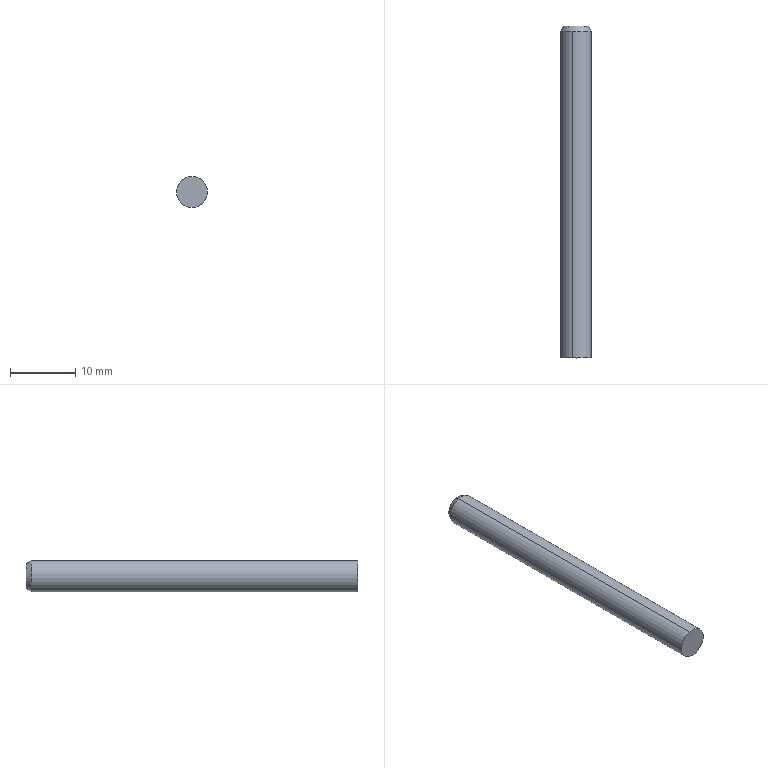Component | SolidWorks | Imported2-1 | 1 solid | 6 faces | box 4.75 x 50.8 x 4.75 mm | volume 898 mm3 | cone 2 | cylinder 2 | plane 2 | commonest cylinder face diameters 4.75 x2
STEP:
#1=CARTESIAN_POINT('',(-8.215,7.373,9.956));
#2=VERTEX_POINT('',#1);
#3=CARTESIAN_POINT('',(-8.178,7.373,9.809));
#4=VERTEX_POINT('',#3);
#5=CARTESIAN_POINT('',(-8.196,7.373,9.883));
#6=DIRECTION('',(0.,1.,-0.));
#7=DIRECTION('',(-0.2492,0.,0.9685));
#8=AXIS2_PLACEMENT_3D('',#5,#6,#7);
#9=CIRCLE('',#8,0.07546);
#10=EDGE_CURVE('',#2,#4,#9,.T.);
#11=ORIENTED_EDGE('',*,*,#10,.F.);
#12=CARTESIAN_POINT('',(-8.22,7.342,9.973));
#13=VERTEX_POINT('',#12);
#14=CARTESIAN_POINT('',(-8.215,7.373,9.956));
#15=DIRECTION('',(-0.1246,-0.866,0.4842));
#16=VECTOR('',#15,39.37);
#17=LINE('',#14,#16);
#18=EDGE_CURVE('',#2,#13,#17,.T.);
#19=ORIENTED_EDGE('',*,*,#18,.T.);
#20=CARTESIAN_POINT('',(-8.173,7.342,9.792));
#21=VERTEX_POINT('',#20);
#22=CARTESIAN_POINT('',(-8.196,7.342,9.883));
#23=DIRECTION('',(-0.,-1.,0.));
#24=DIRECTION('',(-0.2492,0.,0.9685));
#25=AXIS2_PLACEMENT_3D('',#22,#23,#24);
#26=CIRCLE('',#25,0.0935);
#27=EDGE_CURVE('',#21,#13,#26,.T.);
#28=ORIENTED_EDGE('',*,*,#27,.F.);
#29=CARTESIAN_POINT('',(-8.178,7.373,9.809));
#30=DIRECTION('',(0.1246,-0.866,-0.4842));
#31=VECTOR('',#30,39.37);
#32=LINE('',#29,#31);
#33=EDGE_CURVE('',#4,#21,#32,.T.);
#34=ORIENTED_EDGE('',*,*,#33,.F.);
#35=EDGE_LOOP('',(#11,#19,#28,#34));
#36=FACE_OUTER_BOUND('',#35,.T.);
#37=CARTESIAN_POINT('',(-8.196,7.373,9.883));
#38=DIRECTION('',(-0.,-1.,0.));
#39=DIRECTION('',(0.2492,0.,-0.9685));
#40=AXIS2_PLACEMENT_3D('',#37,#38,#39);
#41=CONICAL_SURFACE('',#40,0.07546,0.5236);
#42=ADVANCED_FACE('',(#36),#41,.T.);
#43=ORIENTED_EDGE('',*,*,#27,.T.);
#44=CARTESIAN_POINT('',(-8.22,5.373,9.973));
#45=VERTEX_POINT('',#44);
#46=CARTESIAN_POINT('',(-8.22,7.373,9.973));
#47=DIRECTION('',(-0.,-1.,0.));
#48=VECTOR('',#47,39.37);
#49=LINE('',#46,#48);
#50=EDGE_CURVE('',#13,#45,#49,.T.);
#51=ORIENTED_EDGE('',*,*,#50,.T.);
#52=CARTESIAN_POINT('',(-8.173,5.373,9.792));
#53=VERTEX_POINT('',#52);
#54=CARTESIAN_POINT('',(-8.196,5.373,9.883));
#55=DIRECTION('',(0.,1.,-0.));
#56=DIRECTION('',(-0.2492,0.,0.9685));
#57=AXIS2_PLACEMENT_3D('',#54,#55,#56);
#58=CIRCLE('',#57,0.0935);
#59=EDGE_CURVE('',#45,#53,#58,.T.);
#60=ORIENTED_EDGE('',*,*,#59,.T.);
#61=CARTESIAN_POINT('',(-8.173,7.373,9.792));
#62=DIRECTION('',(-0.,-1.,0.));
#63=VECTOR('',#62,39.37);
#64=LINE('',#61,#63);
#65=EDGE_CURVE('',#21,#53,#64,.T.);
#66=ORIENTED_EDGE('',*,*,#65,.F.);
#67=EDGE_LOOP('',(#43,#51,#60,#66));
#68=FACE_OUTER_BOUND('',#67,.T.);
#69=CARTESIAN_POINT('',(-8.196,7.373,9.883));
#70=DIRECTION('',(-0.,-1.,0.));
#71=DIRECTION('',(0.2492,0.,-0.9685));
#72=AXIS2_PLACEMENT_3D('',#69,#70,#71);
#73=CYLINDRICAL_SURFACE('',#72,0.0935);
#74=ADVANCED_FACE('',(#68),#73,.T.);
#75=ORIENTED_EDGE('',*,*,#50,.F.);
#76=CARTESIAN_POINT('',(-8.196,7.342,9.883));
#77=DIRECTION('',(-0.,-1.,0.));
#78=DIRECTION('',(-0.2492,0.,0.9685));
#79=AXIS2_PLACEMENT_3D('',#76,#77,#78);
#80=CIRCLE('',#79,0.0935);
#81=EDGE_CURVE('',#13,#21,#80,.T.);
#82=ORIENTED_EDGE('',*,*,#81,.T.);
#83=ORIENTED_EDGE('',*,*,#65,.T.);
#84=CARTESIAN_POINT('',(-8.196,5.373,9.883));
#85=DIRECTION('',(0.,1.,-0.));
#86=DIRECTION('',(-0.2492,0.,0.9685));
#87=AXIS2_PLACEMENT_3D('',#84,#85,#86);
#88=CIRCLE('',#87,0.0935);
#89=EDGE_CURVE('',#53,#45,#88,.T.);
#90=ORIENTED_EDGE('',*,*,#89,.T.);
#91=EDGE_LOOP('',(#75,#82,#83,#90));
#92=FACE_OUTER_BOUND('',#91,.T.);
#93=CARTESIAN_POINT('',(-8.196,7.373,9.883));
#94=DIRECTION('',(-0.,-1.,0.));
#95=DIRECTION('',(0.2492,0.,-0.9685));
#96=AXIS2_PLACEMENT_3D('',#93,#94,#95);
#97=CYLINDRICAL_SURFACE('',#96,0.0935);
#98=ADVANCED_FACE('',(#92),#97,.T.);
#99=CARTESIAN_POINT('',(-8.196,7.373,9.883));
#100=DIRECTION('',(0.,1.,-0.));
#101=DIRECTION('',(-0.2492,0.,0.9685));
#102=AXIS2_PLACEMENT_3D('',#99,#100,#101);
#103=CIRCLE('',#102,0.07546);
#104=EDGE_CURVE('',#4,#2,#103,.T.);
#105=ORIENTED_EDGE('',*,*,#104,.T.);
#106=ORIENTED_EDGE('',*,*,#10,.T.);
#107=EDGE_LOOP('',(#105,#106));
#108=FACE_OUTER_BOUND('',#107,.T.);
#109=CARTESIAN_POINT('',(-8.196,7.373,9.883));
#110=DIRECTION('',(0.,1.,0.));
#111=DIRECTION('',(-0.2492,-0.,0.9685));
#112=AXIS2_PLACEMENT_3D('',#109,#110,#111);
#113=PLANE('',#112);
#114=ADVANCED_FACE('',(#108),#113,.T.);
#115=ORIENTED_EDGE('',*,*,#89,.F.);
#116=ORIENTED_EDGE('',*,*,#59,.F.);
#117=EDGE_LOOP('',(#115,#116));
#118=FACE_OUTER_BOUND('',#117,.T.);
#119=CARTESIAN_POINT('',(-8.196,5.373,9.883));
#120=DIRECTION('',(0.,1.,0.));
#121=DIRECTION('',(-0.2492,-0.,0.9685));
#122=AXIS2_PLACEMENT_3D('',#119,#120,#121);
#123=PLANE('',#122);
#124=ADVANCED_FACE('',(#118),#123,.F.);
#125=ORIENTED_EDGE('',*,*,#18,.F.);
#126=ORIENTED_EDGE('',*,*,#104,.F.);
#127=ORIENTED_EDGE('',*,*,#33,.T.);
#128=ORIENTED_EDGE('',*,*,#81,.F.);
#129=EDGE_LOOP('',(#125,#126,#127,#128));
#130=FACE_OUTER_BOUND('',#129,.T.);
#131=CARTESIAN_POINT('',(-8.196,7.373,9.883));
#132=DIRECTION('',(-0.,-1.,0.));
#133=DIRECTION('',(0.2492,0.,-0.9685));
#134=AXIS2_PLACEMENT_3D('',#131,#132,#133);
#135=CONICAL_SURFACE('',#134,0.07546,0.5236);
#136=ADVANCED_FACE('',(#130),#135,.T.);
#137=CLOSED_SHELL('',(#42,#74,#98,#114,#124,#136));
#138=MANIFOLD_SOLID_BREP('',#137);
#139=CARTESIAN_POINT('',(0.,0.,0.));
#140=DIRECTION('',(0.,0.,1.));
#141=DIRECTION('',(1.,0.,0.));
#142=AXIS2_PLACEMENT_3D('',#139,#140,#141);
#143=(LENGTH_UNIT()NAMED_UNIT(*)SI_UNIT($,.METRE.));
#144=LENGTH_MEASURE_WITH_UNIT(LENGTH_MEASURE(0.0254),#143);
#145=DIMENSIONAL_EXPONENTS(1.,0.,0.,0.,0.,0.,0.);
#146=(CONVERSION_BASED_UNIT('',#144)LENGTH_UNIT()NAMED_UNIT(#145));
#147=UNCERTAINTY_MEASURE_WITH_UNIT(LENGTH_MEASURE(0.00001),#146,'','');
#148=(NAMED_UNIT(*)PLANE_ANGLE_UNIT()SI_UNIT($,.RADIAN.));
#149=(NAMED_UNIT(*)SI_UNIT($,.STERADIAN.)SOLID_ANGLE_UNIT());
#150=(GEOMETRIC_REPRESENTATION_CONTEXT(3)GLOBAL_UNCERTAINTY_ASSIGNED_CONTEXT((#147))GLOBAL_UNIT_ASSIGNED_CONTEXT((#146,#148,#149))REPRESENTATION_CONTEXT('',''));
#151=ADVANCED_BREP_SHAPE_REPRESENTATION('',(#138,#142),#150);
#152=COLOUR_RGB('',0.7922,0.8196,0.9333);
#153=FILL_AREA_STYLE_COLOUR('',#152);
#154=FILL_AREA_STYLE('',(#153));
#155=SURFACE_STYLE_FILL_AREA(#154);
#156=SURFACE_SIDE_STYLE('',(#155));
#157=SURFACE_STYLE_USAGE(.BOTH.,#156);
#158=PRESENTATION_STYLE_ASSIGNMENT((#157));
#159=STYLED_ITEM('',(#158),#138);
#160=(LENGTH_UNIT()NAMED_UNIT(*)SI_UNIT($,.METRE.));
#161=LENGTH_MEASURE_WITH_UNIT(LENGTH_MEASURE(0.0254),#160);
#162=DIMENSIONAL_EXPONENTS(1.,0.,0.,0.,0.,0.,0.);
#163=(CONVERSION_BASED_UNIT('',#161)LENGTH_UNIT()NAMED_UNIT(#162));
#164=UNCERTAINTY_MEASURE_WITH_UNIT(LENGTH_MEASURE(0.00001),#163,'','');
#165=(NAMED_UNIT(*)PLANE_ANGLE_UNIT()SI_UNIT($,.RADIAN.));
#166=(NAMED_UNIT(*)SI_UNIT($,.STERADIAN.)SOLID_ANGLE_UNIT());
#167=(GEOMETRIC_REPRESENTATION_CONTEXT(3)GLOBAL_UNCERTAINTY_ASSIGNED_CONTEXT((#164))GLOBAL_UNIT_ASSIGNED_CONTEXT((#163,#165,#166))REPRESENTATION_CONTEXT('',''));
#168=MECHANICAL_DESIGN_GEOMETRIC_PRESENTATION_REPRESENTATION('',(#159),#167);
#169=PRESENTATION_LAYER_ASSIGNMENT('','',(#159));